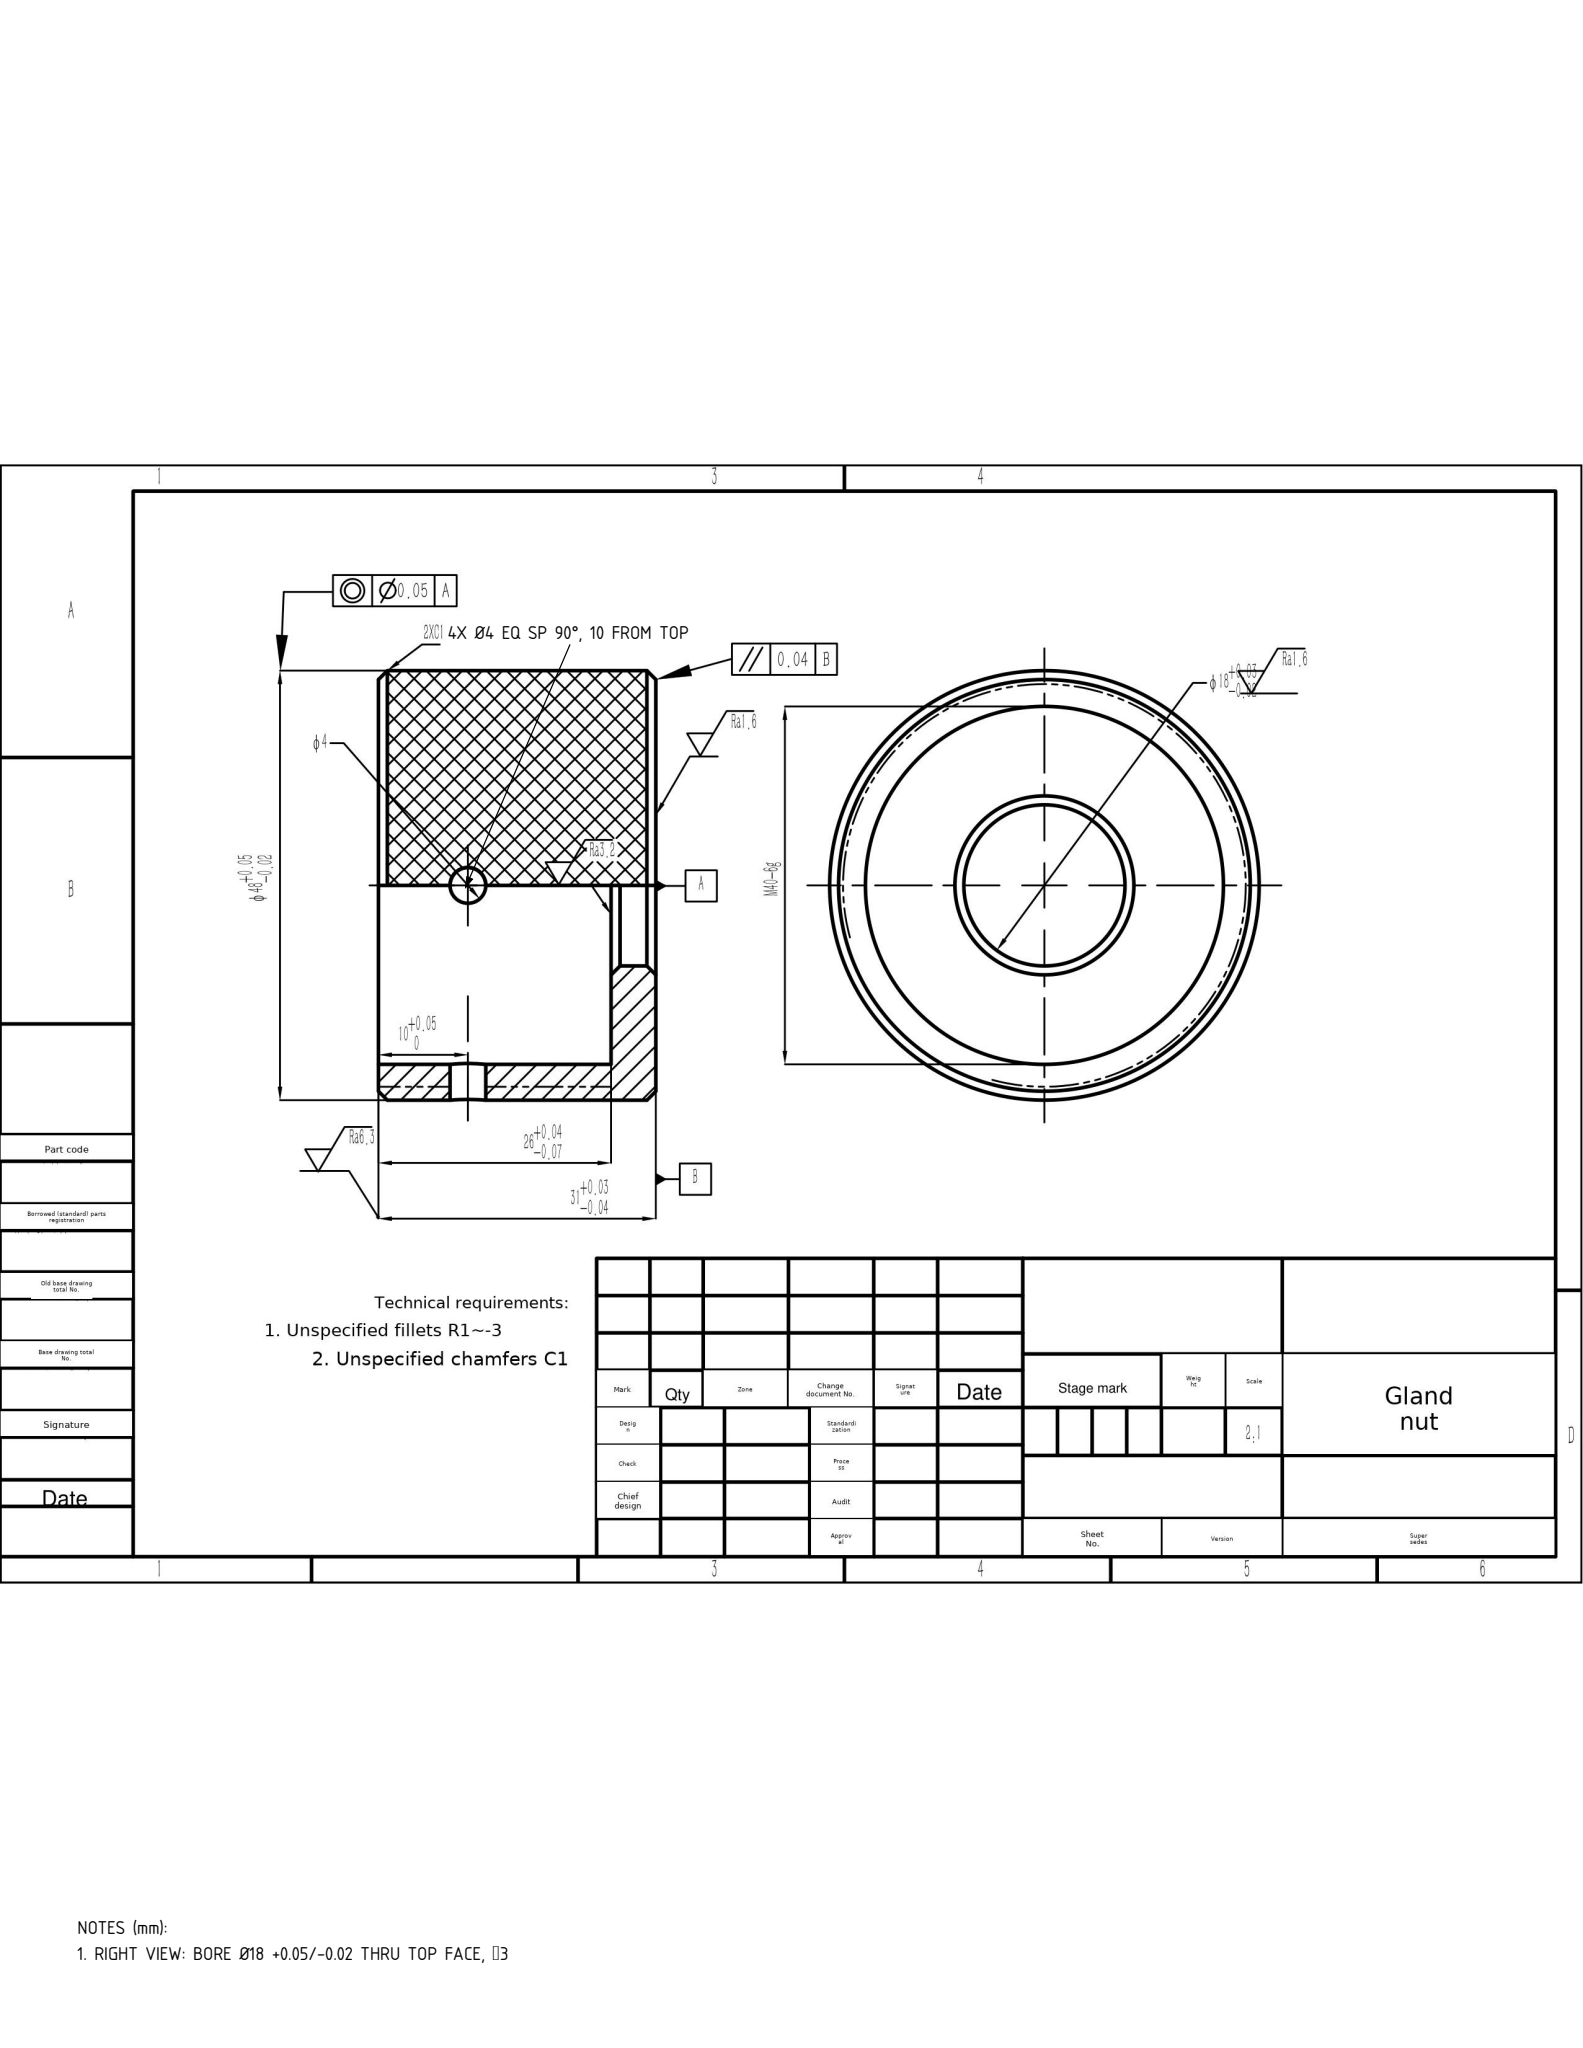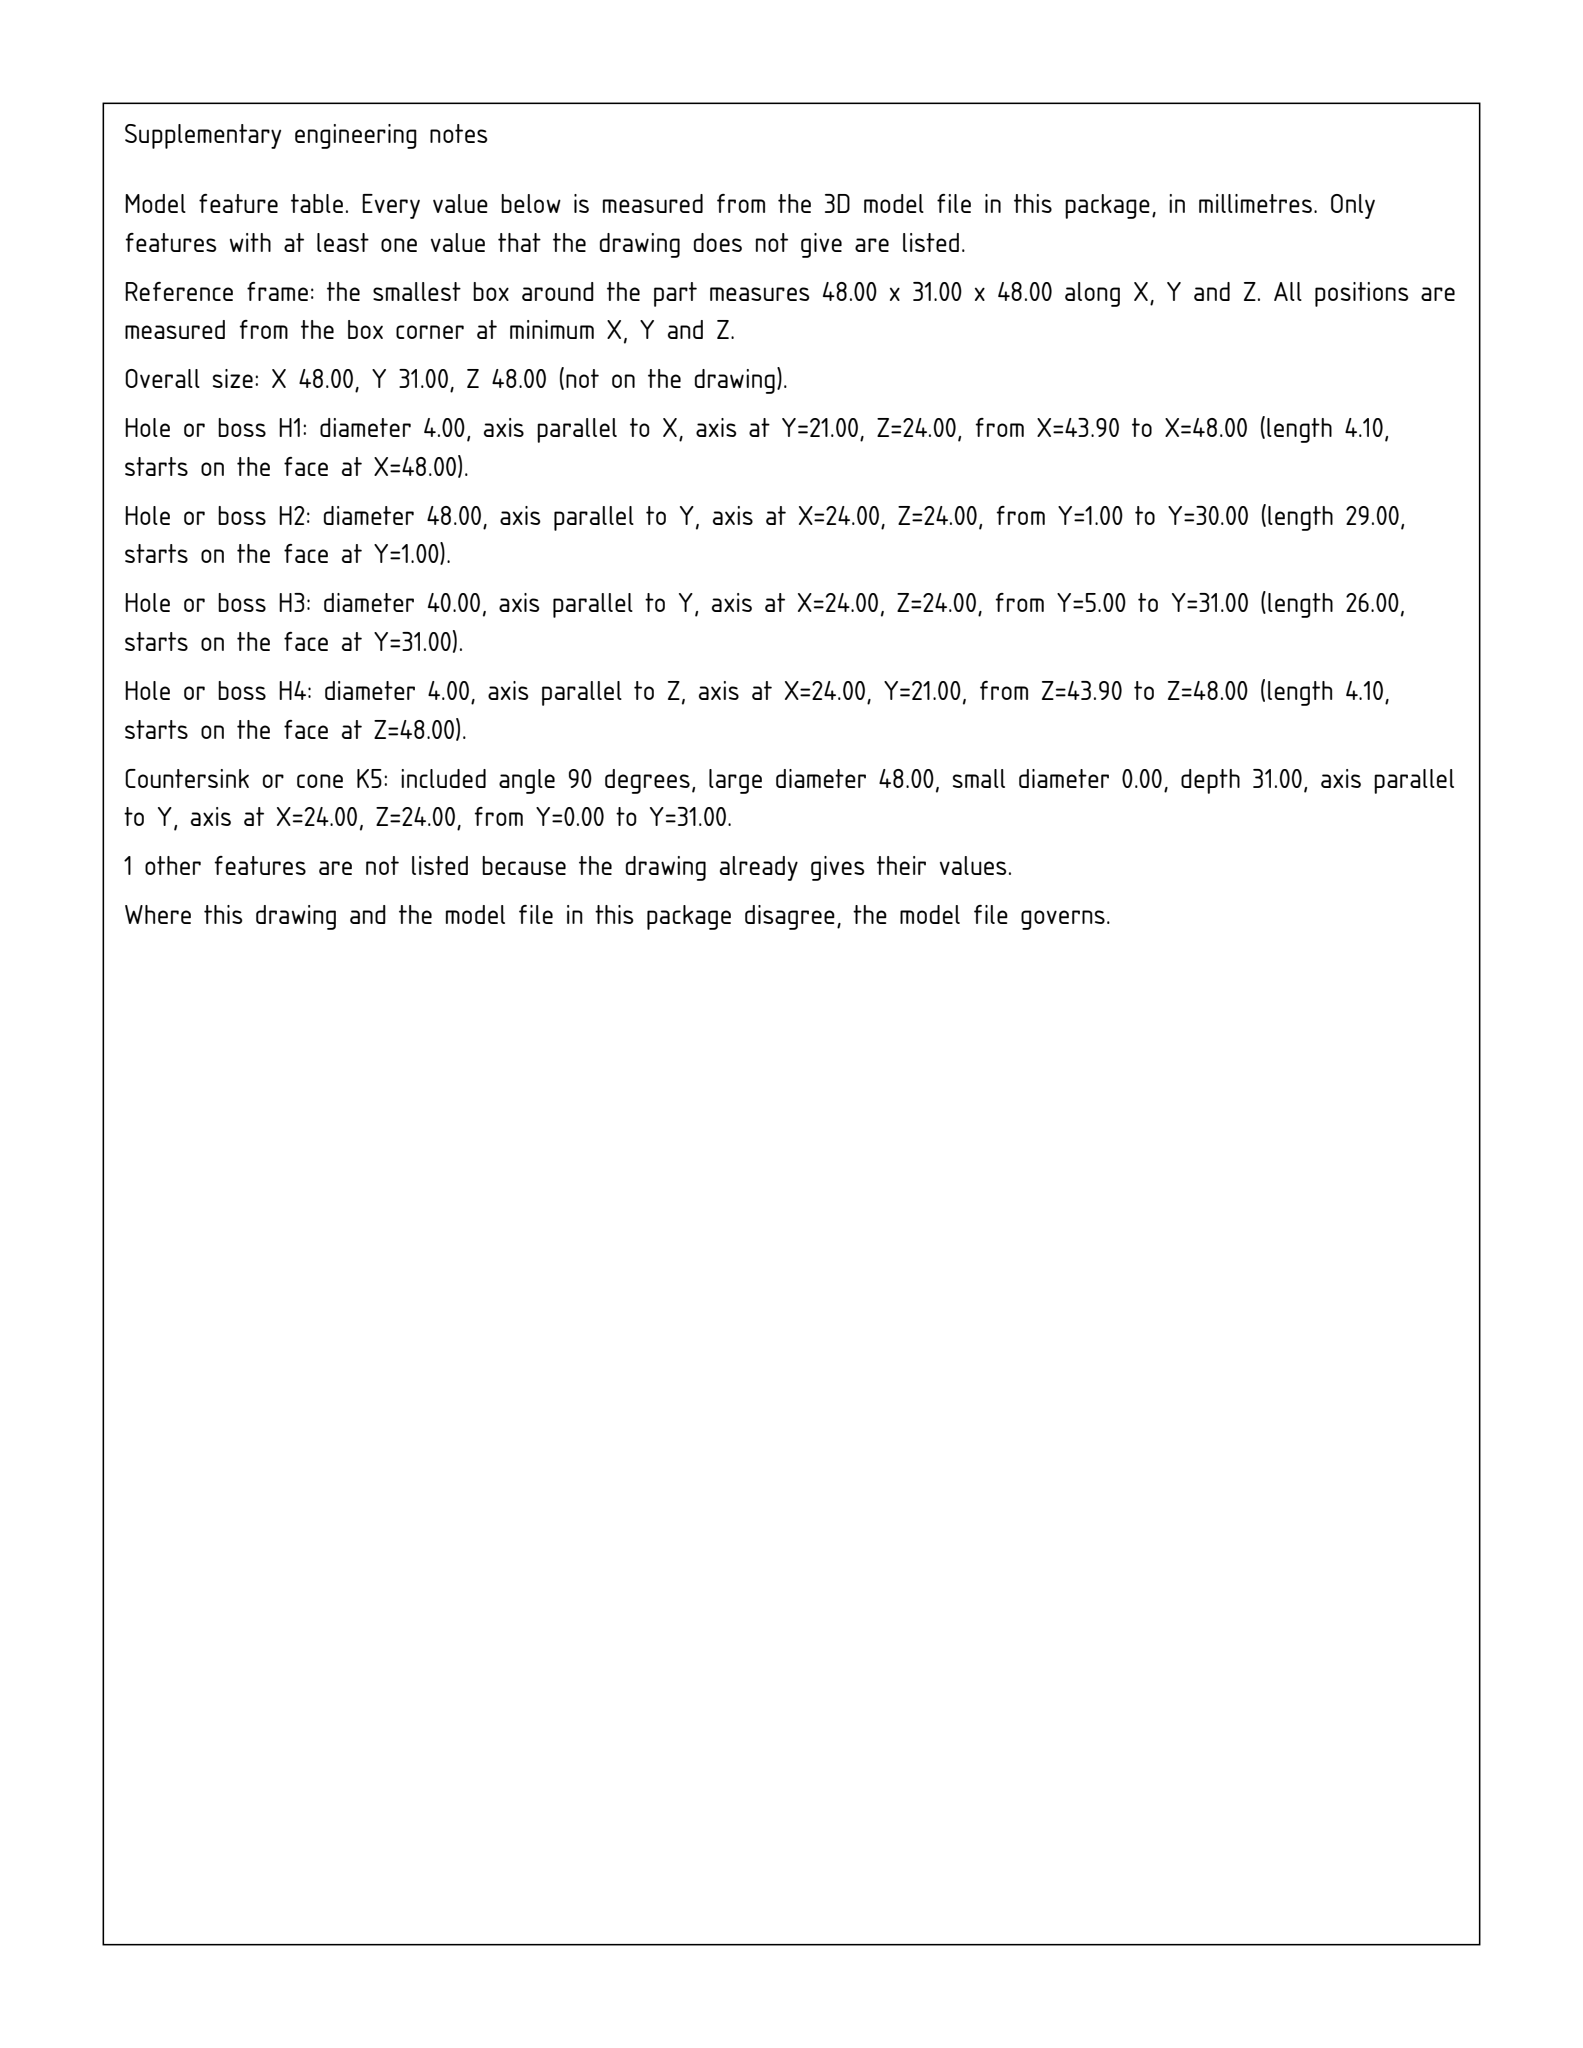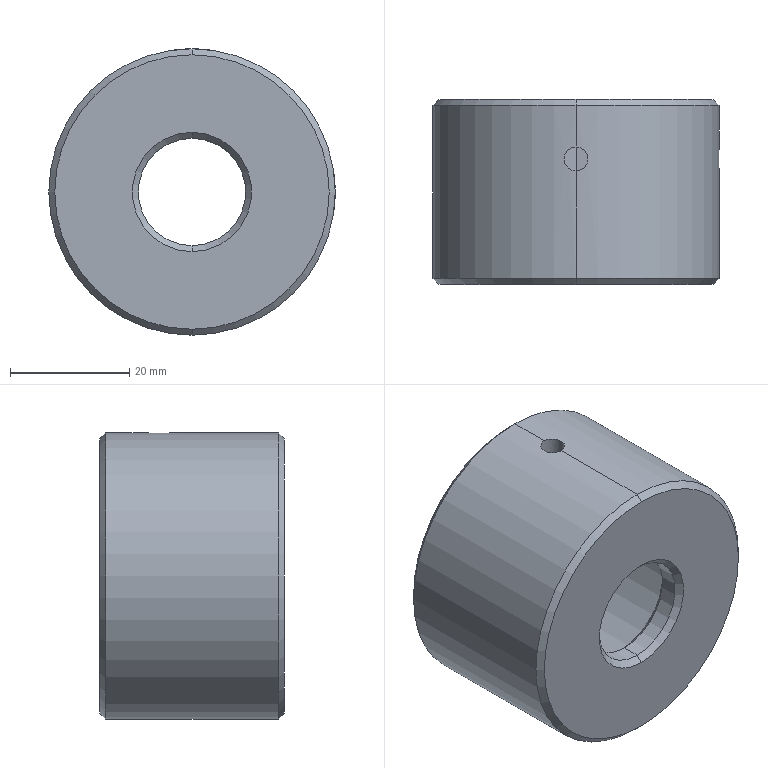Part | SolidWorks | mm | 1 solid | 21 faces | box 48 x 31 x 48 mm | volume 21843 mm3 | cylinder 10 | cone 8 | plane 3 | commonest cylinder face diameters 4 x4 18 x2 40 x2 48 x2
Drawing notes:
4X Ø4 THRU WALL, EQ SP 90°, 10 FROM TOP FACE | from the solid: [4.0,"x",[null,21.0,24.0],4.1,2] + [4.0,"z",[24.0,21.0,null],4.1,2] = 4 radial holes on X and Z axes (90° apart) at y=21; bbox y=31 so 31-21=10 from top face; L=4.1 thru Ø40/Ø48 wall
RIGHT VIEW: BORE Ø18 +0.05/-0.02 THRU TOP FACE, ⅂3 | from the solid: hole/bore dia 18.0 axis y at (24,24), from y=1.0 to 4.0 (3 deep)
build123d program:
from build123d import *

# Parameters (mm, degrees)
SKETCH1_R            = 24
BOSS_EXTRUDE1_DEPTH  = 31
SKETCH2_R            = 20
CUT_EXTRUDE1_DEPTH   = 26
CHAMFER1_SIZE        = 1
SKETCH3_R            = 9
CUT_EXTRUDE2_DEPTH   = 26
CHAMFER2_SIZE        = 1
CUT_SWEEP1_PROFILE_R = 2
CUT_SWEEP2_PROFILE_R = 2


with BuildPart() as part:
    # Sketch1 → Boss-Extrude1 (new body)
    with BuildSketch(Plane(origin=(0, 0, 0), x_dir=(1, 0, 0), z_dir=(0, 1, 0))):
        with Locations(Location((0, 0, 0), (0, 0, 270))):
            Circle(SKETCH1_R)
    extrude(amount=BOSS_EXTRUDE1_DEPTH)

    # Sketch2 → Cut-Extrude1 (cut)
    with BuildSketch(Plane(origin=(0, 31, 0), x_dir=(1, 0, 0), z_dir=(0, 1, 0))):
        with Locations(Location((0, 0, 0), (0, 0, 270))):
            Circle(SKETCH2_R)
    extrude(amount=-CUT_EXTRUDE1_DEPTH, mode=Mode.SUBTRACT)

    # Chamfer1
    chamfer1_edges = [part.edges().sort_by_distance(p)[0] for p in [
        (0, 0, -24),
        (0, 31, -24),
    ]]
    chamfer(chamfer1_edges, length=CHAMFER1_SIZE)

    # Sketch3 → Cut-Extrude2 (cut)
    with BuildSketch(Plane.XZ):
        with Locations(Location((0, 0, 0), (0, 0, 270))):
            Circle(SKETCH3_R)
    extrude(amount=-CUT_EXTRUDE2_DEPTH, mode=Mode.SUBTRACT)

    # Chamfer2
    chamfer2_edges = [part.edges().sort_by_distance(p)[0] for p in [
        (0, 5, 9),
        (0, 0, 9),
    ]]
    chamfer(chamfer2_edges, length=CHAMFER2_SIZE)

    # Cut-Sweep1: sweep along a path in Sketch4
    with BuildLine(Plane.XY) as cut_sweep1_path:
        Line((26.749, 21), (16.823, 21))
    # Cut-Sweep1 profile (on start of the path) → Cut-Sweep1 (sweep, cut)
    with BuildSketch(Plane(origin=(26.749, 21, 0), x_dir=(0, 0, -1), z_dir=(-1, 0, 0))):
        Circle(CUT_SWEEP1_PROFILE_R)
    sweep(path=cut_sweep1_path.line, mode=Mode.SUBTRACT)

    # Cut-Sweep2: sweep along a path in Sketch15
    with BuildLine(Plane(origin=(0, 0, 0), x_dir=(0, 0, -1), z_dir=(1, 0, 0))) as cut_sweep2_path:
        Line((-25.297, 21), (-13.37, 21))
    # Cut-Sweep2 profile (on start of the path) → Cut-Sweep2 (sweep, cut)
    with BuildSketch(Plane(origin=(0, 21, 25.297), x_dir=(-1, 0, 0), z_dir=(0, 0, -1))):
        Circle(CUT_SWEEP2_PROFILE_R)
    sweep(path=cut_sweep2_path.line, mode=Mode.SUBTRACT)


solid = part.part